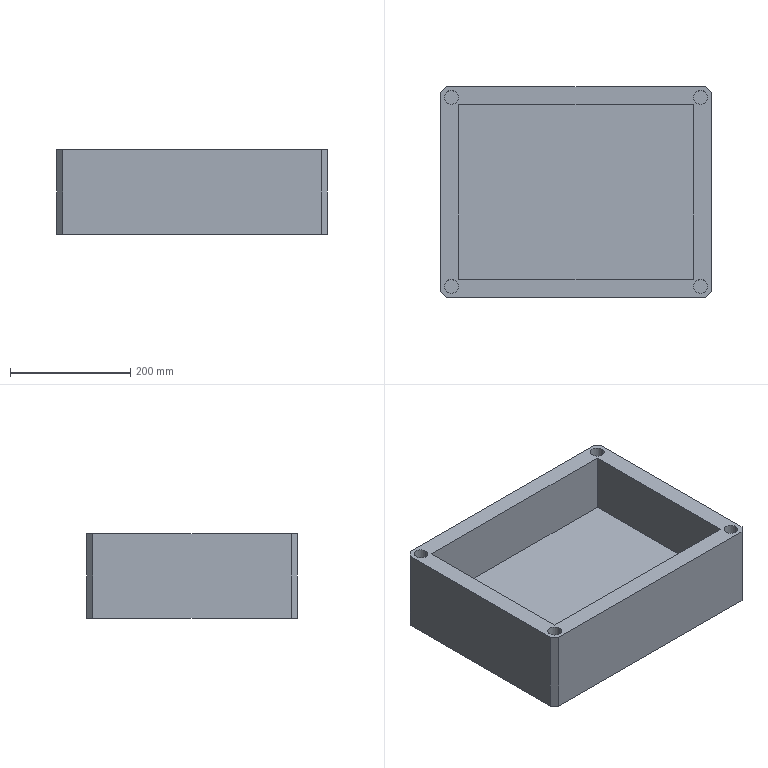Component | SolidWorks | AD12-SquareCellJig.SDPRT-1 | 1 solid | 27 faces | box 450 x 350 x 140 mm | volume 10562429 mm3 | plane 19 | cylinder 8 | commonest cylinder face diameters 23 x8 | material 6061-T6 (SS)
build123d program:
from build123d import *

# Parameters (mm, degrees)
SKETCH1_W           = 450
SKETCH1_H           = 350
BOSS_EXTRUDE1_DEPTH = 140
SKETCH2_W           = 390
SKETCH2_H           = 290
CUT_EXTRUDE1_DEPTH  = 100
SKETCH3_R           = 11.5
CUT_EXTRUDE2_DEPTH  = 90
CHAMFER1_SIZE       = 10


with BuildPart() as part:
    # Sketch1 → Boss-Extrude1 (new body)
    with BuildSketch(Plane.XY):
        Rectangle(SKETCH1_W, SKETCH1_H)
    extrude(amount=BOSS_EXTRUDE1_DEPTH)

    # Sketch2 → Cut-Extrude1 (cut)
    with BuildSketch(Plane.XY.offset(140)):
        Rectangle(SKETCH2_W, SKETCH2_H)
    extrude(amount=-CUT_EXTRUDE1_DEPTH, mode=Mode.SUBTRACT)

    # Sketch3 → Cut-Extrude2 (cut)
    with BuildSketch(Plane.XY.offset(140)):
        with Locations((-207, 157)):
            Circle(SKETCH3_R)
        with Locations((207, 157)):
            Circle(SKETCH3_R)
        with Locations((-207, -157)):
            Circle(SKETCH3_R)
        with Locations((207, -157)):
            Circle(SKETCH3_R)
    extrude(amount=-CUT_EXTRUDE2_DEPTH, mode=Mode.SUBTRACT)

    # Chamfer1
    chamfer1_edges = [part.edges().sort_by_distance(p)[0] for p in [
        (-225, 175, 70),
        (225, 175, 70),
        (225, -175, 70),
        (-225, -175, 70),
    ]]
    chamfer(chamfer1_edges, length=CHAMFER1_SIZE)


solid = part.part

# Placed as in the assembly
solid = solid.moved(Location((-179.414, -13.961, 159.12), (0, 0, 0)))
STEP:
#1=COLOUR_RGB('',0.7922,0.8196,0.9333);
#2=FILL_AREA_STYLE_COLOUR('',#1);
#3=FILL_AREA_STYLE('',(#2));
#4=SURFACE_STYLE_FILL_AREA(#3);
#5=SURFACE_SIDE_STYLE('',(#4));
#6=SURFACE_STYLE_USAGE(.BOTH.,#5);
#7=PRESENTATION_STYLE_ASSIGNMENT((#6));
#8=CARTESIAN_POINT('',(0.6333,-6.731,8.233));
#9=VERTEX_POINT('',#8);
#10=CARTESIAN_POINT('',(1.539,-6.731,8.233));
#11=VERTEX_POINT('',#10);
#12=CARTESIAN_POINT('',(1.086,-6.731,8.233));
#13=DIRECTION('',(0.,0.,1.));
#14=DIRECTION('',(1.,0.,0.));
#15=AXIS2_PLACEMENT_3D('',#12,#13,#14);
#16=CIRCLE('',#15,0.4528);
#17=EDGE_CURVE('',#9,#11,#16,.T.);
#18=ORIENTED_EDGE('',*,*,#17,.F.);
#19=CARTESIAN_POINT('',(0.6333,-6.731,11.776));
#20=VERTEX_POINT('',#19);
#21=CARTESIAN_POINT('',(0.6333,-6.731,8.233));
#22=DIRECTION('',(0.,0.,1.));
#23=VECTOR('',#22,39.37);
#24=LINE('',#21,#23);
#25=EDGE_CURVE('',#9,#20,#24,.T.);
#26=ORIENTED_EDGE('',*,*,#25,.T.);
#27=CARTESIAN_POINT('',(1.539,-6.731,11.776));
#28=VERTEX_POINT('',#27);
#29=CARTESIAN_POINT('',(1.086,-6.731,11.776));
#30=DIRECTION('',(0.,0.,1.));
#31=DIRECTION('',(1.,0.,0.));
#32=AXIS2_PLACEMENT_3D('',#29,#30,#31);
#33=CIRCLE('',#32,0.4528);
#34=EDGE_CURVE('',#20,#28,#33,.T.);
#35=ORIENTED_EDGE('',*,*,#34,.T.);
#36=CARTESIAN_POINT('',(1.539,-6.731,8.233));
#37=DIRECTION('',(0.,0.,1.));
#38=VECTOR('',#37,39.37);
#39=LINE('',#36,#38);
#40=EDGE_CURVE('',#11,#28,#39,.T.);
#41=ORIENTED_EDGE('',*,*,#40,.F.);
#42=EDGE_LOOP('',(#18,#26,#35,#41));
#43=FACE_OUTER_BOUND('',#42,.T.);
#44=CARTESIAN_POINT('',(1.086,-6.731,8.233));
#45=DIRECTION('',(0.,0.,1.));
#46=DIRECTION('',(1.,0.,0.));
#47=AXIS2_PLACEMENT_3D('',#44,#45,#46);
#48=CYLINDRICAL_SURFACE('',#47,0.4528);
#49=ADVANCED_FACE('',(#43),#48,.F.);
#50=CARTESIAN_POINT('',(-15.666,-6.731,8.233));
#51=VERTEX_POINT('',#50);
#52=CARTESIAN_POINT('',(-14.76,-6.731,8.233));
#53=VERTEX_POINT('',#52);
#54=CARTESIAN_POINT('',(-15.213,-6.731,8.233));
#55=DIRECTION('',(0.,0.,1.));
#56=DIRECTION('',(1.,0.,0.));
#57=AXIS2_PLACEMENT_3D('',#54,#55,#56);
#58=CIRCLE('',#57,0.4528);
#59=EDGE_CURVE('',#51,#53,#58,.T.);
#60=ORIENTED_EDGE('',*,*,#59,.F.);
#61=CARTESIAN_POINT('',(-15.666,-6.731,11.776));
#62=VERTEX_POINT('',#61);
#63=CARTESIAN_POINT('',(-15.666,-6.731,8.233));
#64=DIRECTION('',(0.,0.,1.));
#65=VECTOR('',#64,39.37);
#66=LINE('',#63,#65);
#67=EDGE_CURVE('',#51,#62,#66,.T.);
#68=ORIENTED_EDGE('',*,*,#67,.T.);
#69=CARTESIAN_POINT('',(-14.76,-6.731,11.776));
#70=VERTEX_POINT('',#69);
#71=CARTESIAN_POINT('',(-15.213,-6.731,11.776));
#72=DIRECTION('',(0.,0.,1.));
#73=DIRECTION('',(1.,0.,0.));
#74=AXIS2_PLACEMENT_3D('',#71,#72,#73);
#75=CIRCLE('',#74,0.4528);
#76=EDGE_CURVE('',#62,#70,#75,.T.);
#77=ORIENTED_EDGE('',*,*,#76,.T.);
#78=CARTESIAN_POINT('',(-14.76,-6.731,8.233));
#79=DIRECTION('',(0.,0.,1.));
#80=VECTOR('',#79,39.37);
#81=LINE('',#78,#80);
#82=EDGE_CURVE('',#53,#70,#81,.T.);
#83=ORIENTED_EDGE('',*,*,#82,.F.);
#84=EDGE_LOOP('',(#60,#68,#77,#83));
#85=FACE_OUTER_BOUND('',#84,.T.);
#86=CARTESIAN_POINT('',(-15.213,-6.731,8.233));
#87=DIRECTION('',(0.,0.,1.));
#88=DIRECTION('',(1.,0.,0.));
#89=AXIS2_PLACEMENT_3D('',#86,#87,#88);
#90=CYLINDRICAL_SURFACE('',#89,0.4528);
#91=ADVANCED_FACE('',(#85),#90,.F.);
#92=CARTESIAN_POINT('',(0.6333,5.631,8.233));
#93=VERTEX_POINT('',#92);
#94=CARTESIAN_POINT('',(1.539,5.631,8.233));
#95=VERTEX_POINT('',#94);
#96=CARTESIAN_POINT('',(1.086,5.631,8.233));
#97=DIRECTION('',(0.,0.,1.));
#98=DIRECTION('',(1.,0.,0.));
#99=AXIS2_PLACEMENT_3D('',#96,#97,#98);
#100=CIRCLE('',#99,0.4528);
#101=EDGE_CURVE('',#93,#95,#100,.T.);
#102=ORIENTED_EDGE('',*,*,#101,.F.);
#103=CARTESIAN_POINT('',(0.6333,5.631,11.776));
#104=VERTEX_POINT('',#103);
#105=CARTESIAN_POINT('',(0.6333,5.631,8.233));
#106=DIRECTION('',(0.,0.,1.));
#107=VECTOR('',#106,39.37);
#108=LINE('',#105,#107);
#109=EDGE_CURVE('',#93,#104,#108,.T.);
#110=ORIENTED_EDGE('',*,*,#109,.T.);
#111=CARTESIAN_POINT('',(1.539,5.631,11.776));
#112=VERTEX_POINT('',#111);
#113=CARTESIAN_POINT('',(1.086,5.631,11.776));
#114=DIRECTION('',(0.,0.,1.));
#115=DIRECTION('',(1.,0.,0.));
#116=AXIS2_PLACEMENT_3D('',#113,#114,#115);
#117=CIRCLE('',#116,0.4528);
#118=EDGE_CURVE('',#104,#112,#117,.T.);
#119=ORIENTED_EDGE('',*,*,#118,.T.);
#120=CARTESIAN_POINT('',(1.539,5.631,8.233));
#121=DIRECTION('',(0.,0.,1.));
#122=VECTOR('',#121,39.37);
#123=LINE('',#120,#122);
#124=EDGE_CURVE('',#95,#112,#123,.T.);
#125=ORIENTED_EDGE('',*,*,#124,.F.);
#126=EDGE_LOOP('',(#102,#110,#119,#125));
#127=FACE_OUTER_BOUND('',#126,.T.);
#128=CARTESIAN_POINT('',(1.086,5.631,8.233));
#129=DIRECTION('',(0.,0.,1.));
#130=DIRECTION('',(1.,0.,0.));
#131=AXIS2_PLACEMENT_3D('',#128,#129,#130);
#132=CYLINDRICAL_SURFACE('',#131,0.4528);
#133=ADVANCED_FACE('',(#127),#132,.F.);
#134=CARTESIAN_POINT('',(-15.666,5.631,8.233));
#135=VERTEX_POINT('',#134);
#136=CARTESIAN_POINT('',(-14.76,5.631,8.233));
#137=VERTEX_POINT('',#136);
#138=CARTESIAN_POINT('',(-15.213,5.631,8.233));
#139=DIRECTION('',(0.,0.,1.));
#140=DIRECTION('',(1.,0.,0.));
#141=AXIS2_PLACEMENT_3D('',#138,#139,#140);
#142=CIRCLE('',#141,0.4528);
#143=EDGE_CURVE('',#135,#137,#142,.T.);
#144=ORIENTED_EDGE('',*,*,#143,.F.);
#145=CARTESIAN_POINT('',(-15.666,5.631,11.776));
#146=VERTEX_POINT('',#145);
#147=CARTESIAN_POINT('',(-15.666,5.631,8.233));
#148=DIRECTION('',(0.,0.,1.));
#149=VECTOR('',#148,39.37);
#150=LINE('',#147,#149);
#151=EDGE_CURVE('',#135,#146,#150,.T.);
#152=ORIENTED_EDGE('',*,*,#151,.T.);
#153=CARTESIAN_POINT('',(-14.76,5.631,11.776));
#154=VERTEX_POINT('',#153);
#155=CARTESIAN_POINT('',(-15.213,5.631,11.776));
#156=DIRECTION('',(0.,0.,1.));
#157=DIRECTION('',(1.,0.,0.));
#158=AXIS2_PLACEMENT_3D('',#155,#156,#157);
#159=CIRCLE('',#158,0.4528);
#160=EDGE_CURVE('',#146,#154,#159,.T.);
#161=ORIENTED_EDGE('',*,*,#160,.T.);
#162=CARTESIAN_POINT('',(-14.76,5.631,8.233));
#163=DIRECTION('',(0.,0.,1.));
#164=VECTOR('',#163,39.37);
#165=LINE('',#162,#164);
#166=EDGE_CURVE('',#137,#154,#165,.T.);
#167=ORIENTED_EDGE('',*,*,#166,.F.);
#168=EDGE_LOOP('',(#144,#152,#161,#167));
#169=FACE_OUTER_BOUND('',#168,.T.);
#170=CARTESIAN_POINT('',(-15.213,5.631,8.233));
#171=DIRECTION('',(0.,0.,1.));
#172=DIRECTION('',(1.,0.,0.));
#173=AXIS2_PLACEMENT_3D('',#170,#171,#172);
#174=CYLINDRICAL_SURFACE('',#173,0.4528);
#175=ADVANCED_FACE('',(#169),#174,.F.);
#176=CARTESIAN_POINT('',(-15.922,5.946,11.776));
#177=VERTEX_POINT('',#176);
#178=CARTESIAN_POINT('',(-15.922,-7.046,11.776));
#179=VERTEX_POINT('',#178);
#180=CARTESIAN_POINT('',(-15.922,-7.439,11.776));
#181=DIRECTION('',(-0.,-1.,0.));
#182=VECTOR('',#181,39.37);
#183=LINE('',#180,#182);
#184=EDGE_CURVE('',#177,#179,#183,.T.);
#185=ORIENTED_EDGE('',*,*,#184,.F.);
#186=CARTESIAN_POINT('',(-15.922,5.946,6.265));
#187=VERTEX_POINT('',#186);
#188=CARTESIAN_POINT('',(-15.922,5.946,11.776));
#189=DIRECTION('',(0.,0.,-1.));
#190=VECTOR('',#189,39.37);
#191=LINE('',#188,#190);
#192=EDGE_CURVE('',#177,#187,#191,.T.);
#193=ORIENTED_EDGE('',*,*,#192,.T.);
#194=CARTESIAN_POINT('',(-15.922,-7.046,6.265));
#195=VERTEX_POINT('',#194);
#196=CARTESIAN_POINT('',(-15.922,-7.439,6.265));
#197=DIRECTION('',(-0.,-1.,0.));
#198=VECTOR('',#197,39.37);
#199=LINE('',#196,#198);
#200=EDGE_CURVE('',#187,#195,#199,.T.);
#201=ORIENTED_EDGE('',*,*,#200,.T.);
#202=CARTESIAN_POINT('',(-15.922,-7.046,11.776));
#203=DIRECTION('',(0.,0.,1.));
#204=VECTOR('',#203,39.37);
#205=LINE('',#202,#204);
#206=EDGE_CURVE('',#195,#179,#205,.T.);
#207=ORIENTED_EDGE('',*,*,#206,.T.);
#208=EDGE_LOOP('',(#185,#193,#201,#207));
#209=FACE_OUTER_BOUND('',#208,.T.);
#210=CARTESIAN_POINT('',(-15.922,-7.439,11.776));
#211=DIRECTION('',(1.,-0.,0.));
#212=DIRECTION('',(0.,1.,0.));
#213=AXIS2_PLACEMENT_3D('',#210,#211,#212);
#214=PLANE('',#213);
#215=ADVANCED_FACE('',(#209),#214,.F.);
#216=CARTESIAN_POINT('',(-15.528,-7.439,6.265));
#217=VERTEX_POINT('',#216);
#218=CARTESIAN_POINT('',(1.401,-7.439,6.265));
#219=VERTEX_POINT('',#218);
#220=CARTESIAN_POINT('',(-15.922,-7.439,6.265));
#221=DIRECTION('',(1.,0.,0.));
#222=VECTOR('',#221,39.37);
#223=LINE('',#220,#222);
#224=EDGE_CURVE('',#217,#219,#223,.T.);
#225=ORIENTED_EDGE('',*,*,#224,.T.);
#226=CARTESIAN_POINT('',(1.401,-7.439,11.776));
#227=VERTEX_POINT('',#226);
#228=CARTESIAN_POINT('',(1.401,-7.439,11.776));
#229=DIRECTION('',(0.,0.,1.));
#230=VECTOR('',#229,39.37);
#231=LINE('',#228,#230);
#232=EDGE_CURVE('',#219,#227,#231,.T.);
#233=ORIENTED_EDGE('',*,*,#232,.T.);
#234=CARTESIAN_POINT('',(-15.528,-7.439,11.776));
#235=VERTEX_POINT('',#234);
#236=CARTESIAN_POINT('',(-15.922,-7.439,11.776));
#237=DIRECTION('',(1.,0.,0.));
#238=VECTOR('',#237,39.37);
#239=LINE('',#236,#238);
#240=EDGE_CURVE('',#235,#227,#239,.T.);
#241=ORIENTED_EDGE('',*,*,#240,.F.);
#242=CARTESIAN_POINT('',(-15.528,-7.439,11.776));
#243=DIRECTION('',(0.,0.,-1.));
#244=VECTOR('',#243,39.37);
#245=LINE('',#242,#244);
#246=EDGE_CURVE('',#235,#217,#245,.T.);
#247=ORIENTED_EDGE('',*,*,#246,.T.);
#248=EDGE_LOOP('',(#225,#233,#241,#247));
#249=FACE_OUTER_BOUND('',#248,.T.);
#250=CARTESIAN_POINT('',(-15.922,-7.439,11.776));
#251=DIRECTION('',(0.,1.,0.));
#252=DIRECTION('',(0.,0.,1.));
#253=AXIS2_PLACEMENT_3D('',#250,#251,#252);
#254=PLANE('',#253);
#255=ADVANCED_FACE('',(#249),#254,.F.);
#256=CARTESIAN_POINT('',(1.795,-7.046,6.265));
#257=VERTEX_POINT('',#256);
#258=CARTESIAN_POINT('',(1.795,5.946,6.265));
#259=VERTEX_POINT('',#258);
#260=CARTESIAN_POINT('',(1.795,-7.439,6.265));
#261=DIRECTION('',(-0.,1.,0.));
#262=VECTOR('',#261,39.37);
#263=LINE('',#260,#262);
#264=EDGE_CURVE('',#257,#259,#263,.T.);
#265=ORIENTED_EDGE('',*,*,#264,.T.);
#266=CARTESIAN_POINT('',(1.795,5.946,11.776));
#267=VERTEX_POINT('',#266);
#268=CARTESIAN_POINT('',(1.795,5.946,11.776));
#269=DIRECTION('',(0.,0.,1.));
#270=VECTOR('',#269,39.37);
#271=LINE('',#268,#270);
#272=EDGE_CURVE('',#259,#267,#271,.T.);
#273=ORIENTED_EDGE('',*,*,#272,.T.);
#274=CARTESIAN_POINT('',(1.795,-7.046,11.776));
#275=VERTEX_POINT('',#274);
#276=CARTESIAN_POINT('',(1.795,-7.439,11.776));
#277=DIRECTION('',(-0.,1.,0.));
#278=VECTOR('',#277,39.37);
#279=LINE('',#276,#278);
#280=EDGE_CURVE('',#275,#267,#279,.T.);
#281=ORIENTED_EDGE('',*,*,#280,.F.);
#282=CARTESIAN_POINT('',(1.795,-7.046,11.776));
#283=DIRECTION('',(0.,0.,-1.));
#284=VECTOR('',#283,39.37);
#285=LINE('',#282,#284);
#286=EDGE_CURVE('',#275,#257,#285,.T.);
#287=ORIENTED_EDGE('',*,*,#286,.T.);
#288=EDGE_LOOP('',(#265,#273,#281,#287));
#289=FACE_OUTER_BOUND('',#288,.T.);
#290=CARTESIAN_POINT('',(1.795,-7.439,11.776));
#291=DIRECTION('',(-1.,-0.,0.));
#292=DIRECTION('',(0.,-1.,0.));
#293=AXIS2_PLACEMENT_3D('',#290,#291,#292);
#294=PLANE('',#293);
#295=ADVANCED_FACE('',(#289),#294,.F.);
#296=CARTESIAN_POINT('',(1.401,6.34,6.265));
#297=VERTEX_POINT('',#296);
#298=CARTESIAN_POINT('',(-15.528,6.34,6.265));
#299=VERTEX_POINT('',#298);
#300=CARTESIAN_POINT('',(-15.922,6.34,6.265));
#301=DIRECTION('',(-1.,0.,0.));
#302=VECTOR('',#301,39.37);
#303=LINE('',#300,#302);
#304=EDGE_CURVE('',#297,#299,#303,.T.);
#305=ORIENTED_EDGE('',*,*,#304,.T.);
#306=CARTESIAN_POINT('',(-15.528,6.34,11.776));
#307=VERTEX_POINT('',#306);
#308=CARTESIAN_POINT('',(-15.528,6.34,11.776));
#309=DIRECTION('',(0.,0.,1.));
#310=VECTOR('',#309,39.37);
#311=LINE('',#308,#310);
#312=EDGE_CURVE('',#299,#307,#311,.T.);
#313=ORIENTED_EDGE('',*,*,#312,.T.);
#314=CARTESIAN_POINT('',(1.401,6.34,11.776));
#315=VERTEX_POINT('',#314);
#316=CARTESIAN_POINT('',(-15.922,6.34,11.776));
#317=DIRECTION('',(-1.,0.,0.));
#318=VECTOR('',#317,39.37);
#319=LINE('',#316,#318);
#320=EDGE_CURVE('',#315,#307,#319,.T.);
#321=ORIENTED_EDGE('',*,*,#320,.F.);
#322=CARTESIAN_POINT('',(1.401,6.34,11.776));
#323=DIRECTION('',(0.,0.,-1.));
#324=VECTOR('',#323,39.37);
#325=LINE('',#322,#324);
#326=EDGE_CURVE('',#315,#297,#325,.T.);
#327=ORIENTED_EDGE('',*,*,#326,.T.);
#328=EDGE_LOOP('',(#305,#313,#321,#327));
#329=FACE_OUTER_BOUND('',#328,.T.);
#330=CARTESIAN_POINT('',(-15.922,6.34,11.776));
#331=DIRECTION('',(0.,-1.,0.));
#332=DIRECTION('',(0.,0.,-1.));
#333=AXIS2_PLACEMENT_3D('',#330,#331,#332);
#334=PLANE('',#333);
#335=ADVANCED_FACE('',(#329),#334,.F.);
#336=CARTESIAN_POINT('',(1.086,-6.731,11.776));
#337=DIRECTION('',(0.,0.,1.));
#338=DIRECTION('',(1.,0.,0.));
#339=AXIS2_PLACEMENT_3D('',#336,#337,#338);
#340=CIRCLE('',#339,0.4528);
#341=EDGE_CURVE('',#28,#20,#340,.T.);
#342=ORIENTED_EDGE('',*,*,#341,.F.);
#343=ORIENTED_EDGE('',*,*,#34,.F.);
#344=EDGE_LOOP('',(#342,#343));
#345=FACE_BOUND('',#344,.T.);
#346=CARTESIAN_POINT('',(-15.213,-6.731,11.776));
#347=DIRECTION('',(0.,0.,1.));
#348=DIRECTION('',(1.,0.,0.));
#349=AXIS2_PLACEMENT_3D('',#346,#347,#348);
#350=CIRCLE('',#349,0.4528);
#351=EDGE_CURVE('',#70,#62,#350,.T.);
#352=ORIENTED_EDGE('',*,*,#351,.F.);
#353=ORIENTED_EDGE('',*,*,#76,.F.);
#354=EDGE_LOOP('',(#352,#353));
#355=FACE_BOUND('',#354,.T.);
#356=CARTESIAN_POINT('',(1.086,5.631,11.776));
#357=DIRECTION('',(0.,0.,1.));
#358=DIRECTION('',(1.,0.,0.));
#359=AXIS2_PLACEMENT_3D('',#356,#357,#358);
#360=CIRCLE('',#359,0.4528);
#361=EDGE_CURVE('',#112,#104,#360,.T.);
#362=ORIENTED_EDGE('',*,*,#361,.F.);
#363=ORIENTED_EDGE('',*,*,#118,.F.);
#364=EDGE_LOOP('',(#362,#363));
#365=FACE_BOUND('',#364,.T.);
#366=CARTESIAN_POINT('',(-15.213,5.631,11.776));
#367=DIRECTION('',(0.,0.,1.));
#368=DIRECTION('',(1.,0.,0.));
#369=AXIS2_PLACEMENT_3D('',#366,#367,#368);
#370=CIRCLE('',#369,0.4528);
#371=EDGE_CURVE('',#154,#146,#370,.T.);
#372=ORIENTED_EDGE('',*,*,#371,.F.);
#373=ORIENTED_EDGE('',*,*,#160,.F.);
#374=EDGE_LOOP('',(#372,#373));
#375=FACE_BOUND('',#374,.T.);
#376=CARTESIAN_POINT('',(-14.741,-6.258,11.776));
#377=VERTEX_POINT('',#376);
#378=CARTESIAN_POINT('',(0.6136,-6.258,11.776));
#379=VERTEX_POINT('',#378);
#380=CARTESIAN_POINT('',(-14.741,-6.258,11.776));
#381=DIRECTION('',(1.,0.,0.));
#382=VECTOR('',#381,39.37);
#383=LINE('',#380,#382);
#384=EDGE_CURVE('',#377,#379,#383,.T.);
#385=ORIENTED_EDGE('',*,*,#384,.F.);
#386=CARTESIAN_POINT('',(-14.741,5.159,11.776));
#387=VERTEX_POINT('',#386);
#388=CARTESIAN_POINT('',(-14.741,-6.258,11.776));
#389=DIRECTION('',(0.,-1.,0.));
#390=VECTOR('',#389,39.37);
#391=LINE('',#388,#390);
#392=EDGE_CURVE('',#387,#377,#391,.T.);
#393=ORIENTED_EDGE('',*,*,#392,.F.);
#394=CARTESIAN_POINT('',(0.6136,5.159,11.776));
#395=VERTEX_POINT('',#394);
#396=CARTESIAN_POINT('',(-14.741,5.159,11.776));
#397=DIRECTION('',(-1.,-0.,0.));
#398=VECTOR('',#397,39.37);
#399=LINE('',#396,#398);
#400=EDGE_CURVE('',#395,#387,#399,.T.);
#401=ORIENTED_EDGE('',*,*,#400,.F.);
#402=CARTESIAN_POINT('',(0.6136,-6.258,11.776));
#403=DIRECTION('',(-0.,1.,0.));
#404=VECTOR('',#403,39.37);
#405=LINE('',#402,#404);
#406=EDGE_CURVE('',#379,#395,#405,.T.);
#407=ORIENTED_EDGE('',*,*,#406,.F.);
#408=EDGE_LOOP('',(#385,#393,#401,#407));
#409=FACE_BOUND('',#408,.T.);
#410=ORIENTED_EDGE('',*,*,#320,.T.);
#411=CARTESIAN_POINT('',(-15.922,5.946,11.776));
#412=DIRECTION('',(-0.7071,-0.7071,0.));
#413=VECTOR('',#412,39.37);
#414=LINE('',#411,#413);
#415=EDGE_CURVE('',#307,#177,#414,.T.);
#416=ORIENTED_EDGE('',*,*,#415,.T.);
#417=ORIENTED_EDGE('',*,*,#184,.T.);
#418=CARTESIAN_POINT('',(-15.528,-7.439,11.776));
#419=DIRECTION('',(0.7071,-0.7071,0.));
#420=VECTOR('',#419,39.37);
#421=LINE('',#418,#420);
#422=EDGE_CURVE('',#179,#235,#421,.T.);
#423=ORIENTED_EDGE('',*,*,#422,.T.);
#424=ORIENTED_EDGE('',*,*,#240,.T.);
#425=CARTESIAN_POINT('',(1.795,-7.046,11.776));
#426=DIRECTION('',(0.7071,0.7071,0.));
#427=VECTOR('',#426,39.37);
#428=LINE('',#425,#427);
#429=EDGE_CURVE('',#227,#275,#428,.T.);
#430=ORIENTED_EDGE('',*,*,#429,.T.);
#431=ORIENTED_EDGE('',*,*,#280,.T.);
#432=CARTESIAN_POINT('',(1.401,6.34,11.776));
#433=DIRECTION('',(-0.7071,0.7071,0.));
#434=VECTOR('',#433,39.37);
#435=LINE('',#432,#434);
#436=EDGE_CURVE('',#267,#315,#435,.T.);
#437=ORIENTED_EDGE('',*,*,#436,.T.);
#438=EDGE_LOOP('',(#410,#416,#417,#423,#424,#430,#431,#437));
#439=FACE_OUTER_BOUND('',#438,.T.);
#440=CARTESIAN_POINT('',(-7.064,-0.5496,11.776));
#441=DIRECTION('',(0.,0.,-1.));
#442=DIRECTION('',(-1.,0.,0.));
#443=AXIS2_PLACEMENT_3D('',#440,#441,#442);
#444=PLANE('',#443);
#445=ADVANCED_FACE('',(#345,#355,#365,#375,#409,#439),#444,.F.);
#446=ORIENTED_EDGE('',*,*,#200,.F.);
#447=CARTESIAN_POINT('',(-14.741,7.128,6.265));
#448=DIRECTION('',(0.7071,0.7071,0.));
#449=VECTOR('',#448,39.37);
#450=LINE('',#447,#449);
#451=EDGE_CURVE('',#187,#299,#450,.T.);
#452=ORIENTED_EDGE('',*,*,#451,.T.);
#453=ORIENTED_EDGE('',*,*,#304,.F.);
#454=CARTESIAN_POINT('',(0.6136,7.128,6.265));
#455=DIRECTION('',(0.7071,-0.7071,0.));
#456=VECTOR('',#455,39.37);
#457=LINE('',#454,#456);
#458=EDGE_CURVE('',#297,#259,#457,.T.);
#459=ORIENTED_EDGE('',*,*,#458,.T.);
#460=ORIENTED_EDGE('',*,*,#264,.F.);
#461=CARTESIAN_POINT('',(0.6136,-8.227,6.265));
#462=DIRECTION('',(-0.7071,-0.7071,0.));
#463=VECTOR('',#462,39.37);
#464=LINE('',#461,#463);
#465=EDGE_CURVE('',#257,#219,#464,.T.);
#466=ORIENTED_EDGE('',*,*,#465,.T.);
#467=ORIENTED_EDGE('',*,*,#224,.F.);
#468=CARTESIAN_POINT('',(-14.741,-8.227,6.265));
#469=DIRECTION('',(-0.7071,0.7071,0.));
#470=VECTOR('',#469,39.37);
#471=LINE('',#468,#470);
#472=EDGE_CURVE('',#217,#195,#471,.T.);
#473=ORIENTED_EDGE('',*,*,#472,.T.);
#474=EDGE_LOOP('',(#446,#452,#453,#459,#460,#466,#467,#473));
#475=FACE_OUTER_BOUND('',#474,.T.);
#476=CARTESIAN_POINT('',(-7.064,-0.5496,6.265));
#477=DIRECTION('',(0.,0.,-1.));
#478=DIRECTION('',(-1.,0.,0.));
#479=AXIS2_PLACEMENT_3D('',#476,#477,#478);
#480=PLANE('',#479);
#481=ADVANCED_FACE('',(#475),#480,.T.);
#482=ORIENTED_EDGE('',*,*,#392,.T.);
#483=CARTESIAN_POINT('',(-14.741,-6.258,7.839));
#484=VERTEX_POINT('',#483);
#485=CARTESIAN_POINT('',(-14.741,-6.258,7.839));
#486=DIRECTION('',(0.,0.,1.));
#487=VECTOR('',#486,39.37);
#488=LINE('',#485,#487);
#489=EDGE_CURVE('',#484,#377,#488,.T.);
#490=ORIENTED_EDGE('',*,*,#489,.F.);
#491=CARTESIAN_POINT('',(-14.741,5.159,7.839));
#492=VERTEX_POINT('',#491);
#493=CARTESIAN_POINT('',(-14.741,-6.258,7.839));
#494=DIRECTION('',(0.,-1.,0.));
#495=VECTOR('',#494,39.37);
#496=LINE('',#493,#495);
#497=EDGE_CURVE('',#492,#484,#496,.T.);
#498=ORIENTED_EDGE('',*,*,#497,.F.);
#499=CARTESIAN_POINT('',(-14.741,5.159,7.839));
#500=DIRECTION('',(0.,0.,1.));
#501=VECTOR('',#500,39.37);
#502=LINE('',#499,#501);
#503=EDGE_CURVE('',#492,#387,#502,.T.);
#504=ORIENTED_EDGE('',*,*,#503,.T.);
#505=EDGE_LOOP('',(#482,#490,#498,#504));
#506=FACE_OUTER_BOUND('',#505,.T.);
#507=CARTESIAN_POINT('',(-14.741,-6.258,7.839));
#508=DIRECTION('',(-1.,0.,0.));
#509=DIRECTION('',(0.,0.,1.));
#510=AXIS2_PLACEMENT_3D('',#507,#508,#509);
#511=PLANE('',#510);
#512=ADVANCED_FACE('',(#506),#511,.F.);
#513=ORIENTED_EDGE('',*,*,#400,.T.);
#514=ORIENTED_EDGE('',*,*,#503,.F.);
#515=CARTESIAN_POINT('',(0.6136,5.159,7.839));
#516=VERTEX_POINT('',#515);
#517=CARTESIAN_POINT('',(-14.741,5.159,7.839));
#518=DIRECTION('',(-1.,-0.,0.));
#519=VECTOR('',#518,39.37);
#520=LINE('',#517,#519);
#521=EDGE_CURVE('',#516,#492,#520,.T.);
#522=ORIENTED_EDGE('',*,*,#521,.F.);
#523=CARTESIAN_POINT('',(0.6136,5.159,7.839));
#524=DIRECTION('',(0.,0.,1.));
#525=VECTOR('',#524,39.37);
#526=LINE('',#523,#525);
#527=EDGE_CURVE('',#516,#395,#526,.T.);
#528=ORIENTED_EDGE('',*,*,#527,.T.);
#529=EDGE_LOOP('',(#513,#514,#522,#528));
#530=FACE_OUTER_BOUND('',#529,.T.);
#531=CARTESIAN_POINT('',(-14.741,5.159,7.839));
#532=DIRECTION('',(-0.,1.,0.));
#533=DIRECTION('',(-1.,-0.,0.));
#534=AXIS2_PLACEMENT_3D('',#531,#532,#533);
#535=PLANE('',#534);
#536=ADVANCED_FACE('',(#530),#535,.F.);
#537=ORIENTED_EDGE('',*,*,#406,.T.);
#538=ORIENTED_EDGE('',*,*,#527,.F.);
#539=CARTESIAN_POINT('',(0.6136,-6.258,7.839));
#540=VERTEX_POINT('',#539);
#541=CARTESIAN_POINT('',(0.6136,-6.258,7.839));
#542=DIRECTION('',(-0.,1.,0.));
#543=VECTOR('',#542,39.37);
#544=LINE('',#541,#543);
#545=EDGE_CURVE('',#540,#516,#544,.T.);
#546=ORIENTED_EDGE('',*,*,#545,.F.);
#547=CARTESIAN_POINT('',(0.6136,-6.258,7.839));
#548=DIRECTION('',(0.,0.,1.));
#549=VECTOR('',#548,39.37);
#550=LINE('',#547,#549);
#551=EDGE_CURVE('',#540,#379,#550,.T.);
#552=ORIENTED_EDGE('',*,*,#551,.T.);
#553=EDGE_LOOP('',(#537,#538,#546,#552));
#554=FACE_OUTER_BOUND('',#553,.T.);
#555=CARTESIAN_POINT('',(0.6136,-6.258,7.839));
#556=DIRECTION('',(1.,0.,0.));
#557=DIRECTION('',(-0.,1.,0.));
#558=AXIS2_PLACEMENT_3D('',#555,#556,#557);
#559=PLANE('',#558);
#560=ADVANCED_FACE('',(#554),#559,.F.);
#561=ORIENTED_EDGE('',*,*,#384,.T.);
#562=ORIENTED_EDGE('',*,*,#551,.F.);
#563=CARTESIAN_POINT('',(-14.741,-6.258,7.839));
#564=DIRECTION('',(1.,0.,0.));
#565=VECTOR('',#564,39.37);
#566=LINE('',#563,#565);
#567=EDGE_CURVE('',#484,#540,#566,.T.);
#568=ORIENTED_EDGE('',*,*,#567,.F.);
#569=ORIENTED_EDGE('',*,*,#489,.T.);
#570=EDGE_LOOP('',(#561,#562,#568,#569));
#571=FACE_OUTER_BOUND('',#570,.T.);
#572=CARTESIAN_POINT('',(-14.741,-6.258,7.839));
#573=DIRECTION('',(0.,-1.,0.));
#574=DIRECTION('',(0.,0.,-1.));
#575=AXIS2_PLACEMENT_3D('',#572,#573,#574);
#576=PLANE('',#575);
#577=ADVANCED_FACE('',(#571),#576,.F.);
#578=ORIENTED_EDGE('',*,*,#497,.T.);
#579=ORIENTED_EDGE('',*,*,#567,.T.);
#580=ORIENTED_EDGE('',*,*,#545,.T.);
#581=ORIENTED_EDGE('',*,*,#521,.T.);
#582=EDGE_LOOP('',(#578,#579,#580,#581));
#583=FACE_OUTER_BOUND('',#582,.T.);
#584=CARTESIAN_POINT('',(-7.064,-0.5496,7.839));
#585=DIRECTION('',(0.,0.,-1.));
#586=DIRECTION('',(-1.,0.,0.));
#587=AXIS2_PLACEMENT_3D('',#584,#585,#586);
#588=PLANE('',#587);
#589=ADVANCED_FACE('',(#583),#588,.F.);
#590=ORIENTED_EDGE('',*,*,#151,.F.);
#591=CARTESIAN_POINT('',(-15.213,5.631,8.233));
#592=DIRECTION('',(0.,0.,1.));
#593=DIRECTION('',(1.,0.,0.));
#594=AXIS2_PLACEMENT_3D('',#591,#592,#593);
#595=CIRCLE('',#594,0.4528);
#596=EDGE_CURVE('',#137,#135,#595,.T.);
#597=ORIENTED_EDGE('',*,*,#596,.F.);
#598=ORIENTED_EDGE('',*,*,#166,.T.);
#599=ORIENTED_EDGE('',*,*,#371,.T.);
#600=EDGE_LOOP('',(#590,#597,#598,#599));
#601=FACE_OUTER_BOUND('',#600,.T.);
#602=CARTESIAN_POINT('',(-15.213,5.631,8.233));
#603=DIRECTION('',(0.,0.,1.));
#604=DIRECTION('',(1.,0.,0.));
#605=AXIS2_PLACEMENT_3D('',#602,#603,#604);
#606=CYLINDRICAL_SURFACE('',#605,0.4528);
#607=ADVANCED_FACE('',(#601),#606,.F.);
#608=ORIENTED_EDGE('',*,*,#596,.T.);
#609=ORIENTED_EDGE('',*,*,#143,.T.);
#610=EDGE_LOOP('',(#608,#609));
#611=FACE_OUTER_BOUND('',#610,.T.);
#612=CARTESIAN_POINT('',(-15.213,5.631,8.233));
#613=DIRECTION('',(0.,0.,1.));
#614=DIRECTION('',(1.,0.,0.));
#615=AXIS2_PLACEMENT_3D('',#612,#613,#614);
#616=PLANE('',#615);
#617=ADVANCED_FACE('',(#611),#616,.T.);
#618=ORIENTED_EDGE('',*,*,#109,.F.);
#619=CARTESIAN_POINT('',(1.086,5.631,8.233));
#620=DIRECTION('',(0.,0.,1.));
#621=DIRECTION('',(1.,0.,0.));
#622=AXIS2_PLACEMENT_3D('',#619,#620,#621);
#623=CIRCLE('',#622,0.4528);
#624=EDGE_CURVE('',#95,#93,#623,.T.);
#625=ORIENTED_EDGE('',*,*,#624,.F.);
#626=ORIENTED_EDGE('',*,*,#124,.T.);
#627=ORIENTED_EDGE('',*,*,#361,.T.);
#628=EDGE_LOOP('',(#618,#625,#626,#627));
#629=FACE_OUTER_BOUND('',#628,.T.);
#630=CARTESIAN_POINT('',(1.086,5.631,8.233));
#631=DIRECTION('',(0.,0.,1.));
#632=DIRECTION('',(1.,0.,0.));
#633=AXIS2_PLACEMENT_3D('',#630,#631,#632);
#634=CYLINDRICAL_SURFACE('',#633,0.4528);
#635=ADVANCED_FACE('',(#629),#634,.F.);
#636=ORIENTED_EDGE('',*,*,#624,.T.);
#637=ORIENTED_EDGE('',*,*,#101,.T.);
#638=EDGE_LOOP('',(#636,#637));
#639=FACE_OUTER_BOUND('',#638,.T.);
#640=CARTESIAN_POINT('',(1.086,5.631,8.233));
#641=DIRECTION('',(0.,0.,1.));
#642=DIRECTION('',(1.,0.,0.));
#643=AXIS2_PLACEMENT_3D('',#640,#641,#642);
#644=PLANE('',#643);
#645=ADVANCED_FACE('',(#639),#644,.T.);
#646=ORIENTED_EDGE('',*,*,#67,.F.);
#647=CARTESIAN_POINT('',(-15.213,-6.731,8.233));
#648=DIRECTION('',(0.,0.,1.));
#649=DIRECTION('',(1.,0.,0.));
#650=AXIS2_PLACEMENT_3D('',#647,#648,#649);
#651=CIRCLE('',#650,0.4528);
#652=EDGE_CURVE('',#53,#51,#651,.T.);
#653=ORIENTED_EDGE('',*,*,#652,.F.);
#654=ORIENTED_EDGE('',*,*,#82,.T.);
#655=ORIENTED_EDGE('',*,*,#351,.T.);
#656=EDGE_LOOP('',(#646,#653,#654,#655));
#657=FACE_OUTER_BOUND('',#656,.T.);
#658=CARTESIAN_POINT('',(-15.213,-6.731,8.233));
#659=DIRECTION('',(0.,0.,1.));
#660=DIRECTION('',(1.,0.,0.));
#661=AXIS2_PLACEMENT_3D('',#658,#659,#660);
#662=CYLINDRICAL_SURFACE('',#661,0.4528);
#663=ADVANCED_FACE('',(#657),#662,.F.);
#664=ORIENTED_EDGE('',*,*,#652,.T.);
#665=ORIENTED_EDGE('',*,*,#59,.T.);
#666=EDGE_LOOP('',(#664,#665));
#667=FACE_OUTER_BOUND('',#666,.T.);
#668=CARTESIAN_POINT('',(-15.213,-6.731,8.233));
#669=DIRECTION('',(0.,0.,1.));
#670=DIRECTION('',(1.,0.,0.));
#671=AXIS2_PLACEMENT_3D('',#668,#669,#670);
#672=PLANE('',#671);
#673=ADVANCED_FACE('',(#667),#672,.T.);
#674=ORIENTED_EDGE('',*,*,#25,.F.);
#675=CARTESIAN_POINT('',(1.086,-6.731,8.233));
#676=DIRECTION('',(0.,0.,1.));
#677=DIRECTION('',(1.,0.,0.));
#678=AXIS2_PLACEMENT_3D('',#675,#676,#677);
#679=CIRCLE('',#678,0.4528);
#680=EDGE_CURVE('',#11,#9,#679,.T.);
#681=ORIENTED_EDGE('',*,*,#680,.F.);
#682=ORIENTED_EDGE('',*,*,#40,.T.);
#683=ORIENTED_EDGE('',*,*,#341,.T.);
#684=EDGE_LOOP('',(#674,#681,#682,#683));
#685=FACE_OUTER_BOUND('',#684,.T.);
#686=CARTESIAN_POINT('',(1.086,-6.731,8.233));
#687=DIRECTION('',(0.,0.,1.));
#688=DIRECTION('',(1.,0.,0.));
#689=AXIS2_PLACEMENT_3D('',#686,#687,#688);
#690=CYLINDRICAL_SURFACE('',#689,0.4528);
#691=ADVANCED_FACE('',(#685),#690,.F.);
#692=ORIENTED_EDGE('',*,*,#680,.T.);
#693=ORIENTED_EDGE('',*,*,#17,.T.);
#694=EDGE_LOOP('',(#692,#693));
#695=FACE_OUTER_BOUND('',#694,.T.);
#696=CARTESIAN_POINT('',(1.086,-6.731,8.233));
#697=DIRECTION('',(0.,0.,1.));
#698=DIRECTION('',(1.,0.,0.));
#699=AXIS2_PLACEMENT_3D('',#696,#697,#698);
#700=PLANE('',#699);
#701=ADVANCED_FACE('',(#695),#700,.T.);
#702=ORIENTED_EDGE('',*,*,#415,.F.);
#703=ORIENTED_EDGE('',*,*,#312,.F.);
#704=ORIENTED_EDGE('',*,*,#451,.F.);
#705=ORIENTED_EDGE('',*,*,#192,.F.);
#706=EDGE_LOOP('',(#702,#703,#704,#705));
#707=FACE_OUTER_BOUND('',#706,.T.);
#708=CARTESIAN_POINT('',(-15.922,5.946,11.776));
#709=DIRECTION('',(0.7071,-0.7071,0.));
#710=DIRECTION('',(0.,0.,-1.));
#711=AXIS2_PLACEMENT_3D('',#708,#709,#710);
#712=PLANE('',#711);
#713=ADVANCED_FACE('',(#707),#712,.F.);
#714=ORIENTED_EDGE('',*,*,#436,.F.);
#715=ORIENTED_EDGE('',*,*,#272,.F.);
#716=ORIENTED_EDGE('',*,*,#458,.F.);
#717=ORIENTED_EDGE('',*,*,#326,.F.);
#718=EDGE_LOOP('',(#714,#715,#716,#717));
#719=FACE_OUTER_BOUND('',#718,.T.);
#720=CARTESIAN_POINT('',(1.401,6.34,11.776));
#721=DIRECTION('',(-0.7071,-0.7071,0.));
#722=DIRECTION('',(0.,0.,-1.));
#723=AXIS2_PLACEMENT_3D('',#720,#721,#722);
#724=PLANE('',#723);
#725=ADVANCED_FACE('',(#719),#724,.F.);
#726=ORIENTED_EDGE('',*,*,#429,.F.);
#727=ORIENTED_EDGE('',*,*,#232,.F.);
#728=ORIENTED_EDGE('',*,*,#465,.F.);
#729=ORIENTED_EDGE('',*,*,#286,.F.);
#730=EDGE_LOOP('',(#726,#727,#728,#729));
#731=FACE_OUTER_BOUND('',#730,.T.);
#732=CARTESIAN_POINT('',(1.795,-7.046,11.776));
#733=DIRECTION('',(-0.7071,0.7071,0.));
#734=DIRECTION('',(0.,0.,-1.));
#735=AXIS2_PLACEMENT_3D('',#732,#733,#734);
#736=PLANE('',#735);
#737=ADVANCED_FACE('',(#731),#736,.F.);
#738=ORIENTED_EDGE('',*,*,#422,.F.);
#739=ORIENTED_EDGE('',*,*,#206,.F.);
#740=ORIENTED_EDGE('',*,*,#472,.F.);
#741=ORIENTED_EDGE('',*,*,#246,.F.);
#742=EDGE_LOOP('',(#738,#739,#740,#741));
#743=FACE_OUTER_BOUND('',#742,.T.);
#744=CARTESIAN_POINT('',(-15.528,-7.439,11.776));
#745=DIRECTION('',(0.7071,0.7071,0.));
#746=DIRECTION('',(0.,0.,-1.));
#747=AXIS2_PLACEMENT_3D('',#744,#745,#746);
#748=PLANE('',#747);
#749=ADVANCED_FACE('',(#743),#748,.F.);
#750=CLOSED_SHELL('',(#49,#91,#133,#175,#215,#255,#295,#335,#445,#481,#512,#536,#560,#577,#589,#607,#617,#635,#645,#663,#673,#691,#701,#713,#725,#737,#749));
#751=MANIFOLD_SOLID_BREP('',#750);
#752=STYLED_ITEM('',(#7),#751);
#753=PRESENTATION_LAYER_ASSIGNMENT('','',(#752));
#754=(LENGTH_UNIT()NAMED_UNIT(*)SI_UNIT($,.METRE.));
#755=LENGTH_MEASURE_WITH_UNIT(LENGTH_MEASURE(0.0254),#754);
#756=DIMENSIONAL_EXPONENTS(1.,0.,0.,0.,0.,0.,0.);
#757=(CONVERSION_BASED_UNIT('',#755)LENGTH_UNIT()NAMED_UNIT(#756));
#758=UNCERTAINTY_MEASURE_WITH_UNIT(LENGTH_MEASURE(0.00001),#757,'','');
#759=(NAMED_UNIT(*)PLANE_ANGLE_UNIT()SI_UNIT($,.RADIAN.));
#760=(NAMED_UNIT(*)SI_UNIT($,.STERADIAN.)SOLID_ANGLE_UNIT());
#761=(GEOMETRIC_REPRESENTATION_CONTEXT(3)GLOBAL_UNCERTAINTY_ASSIGNED_CONTEXT((#758))GLOBAL_UNIT_ASSIGNED_CONTEXT((#757,#759,#760))REPRESENTATION_CONTEXT('',''));
#762=MECHANICAL_DESIGN_GEOMETRIC_PRESENTATION_REPRESENTATION('',(#752),#761);
#763=CARTESIAN_POINT('',(0.,0.,0.));
#764=DIRECTION('',(0.,0.,1.));
#765=DIRECTION('',(1.,0.,0.));
#766=AXIS2_PLACEMENT_3D('',#763,#764,#765);
#767=(LENGTH_UNIT()NAMED_UNIT(*)SI_UNIT($,.METRE.));
#768=LENGTH_MEASURE_WITH_UNIT(LENGTH_MEASURE(0.0254),#767);
#769=DIMENSIONAL_EXPONENTS(1.,0.,0.,0.,0.,0.,0.);
#770=(CONVERSION_BASED_UNIT('',#768)LENGTH_UNIT()NAMED_UNIT(#769));
#771=UNCERTAINTY_MEASURE_WITH_UNIT(LENGTH_MEASURE(0.00001),#770,'','');
#772=(NAMED_UNIT(*)PLANE_ANGLE_UNIT()SI_UNIT($,.RADIAN.));
#773=(NAMED_UNIT(*)SI_UNIT($,.STERADIAN.)SOLID_ANGLE_UNIT());
#774=(GEOMETRIC_REPRESENTATION_CONTEXT(3)GLOBAL_UNCERTAINTY_ASSIGNED_CONTEXT((#771))GLOBAL_UNIT_ASSIGNED_CONTEXT((#770,#772,#773))REPRESENTATION_CONTEXT('',''));
#775=ADVANCED_BREP_SHAPE_REPRESENTATION('',(#751,#766),#774);